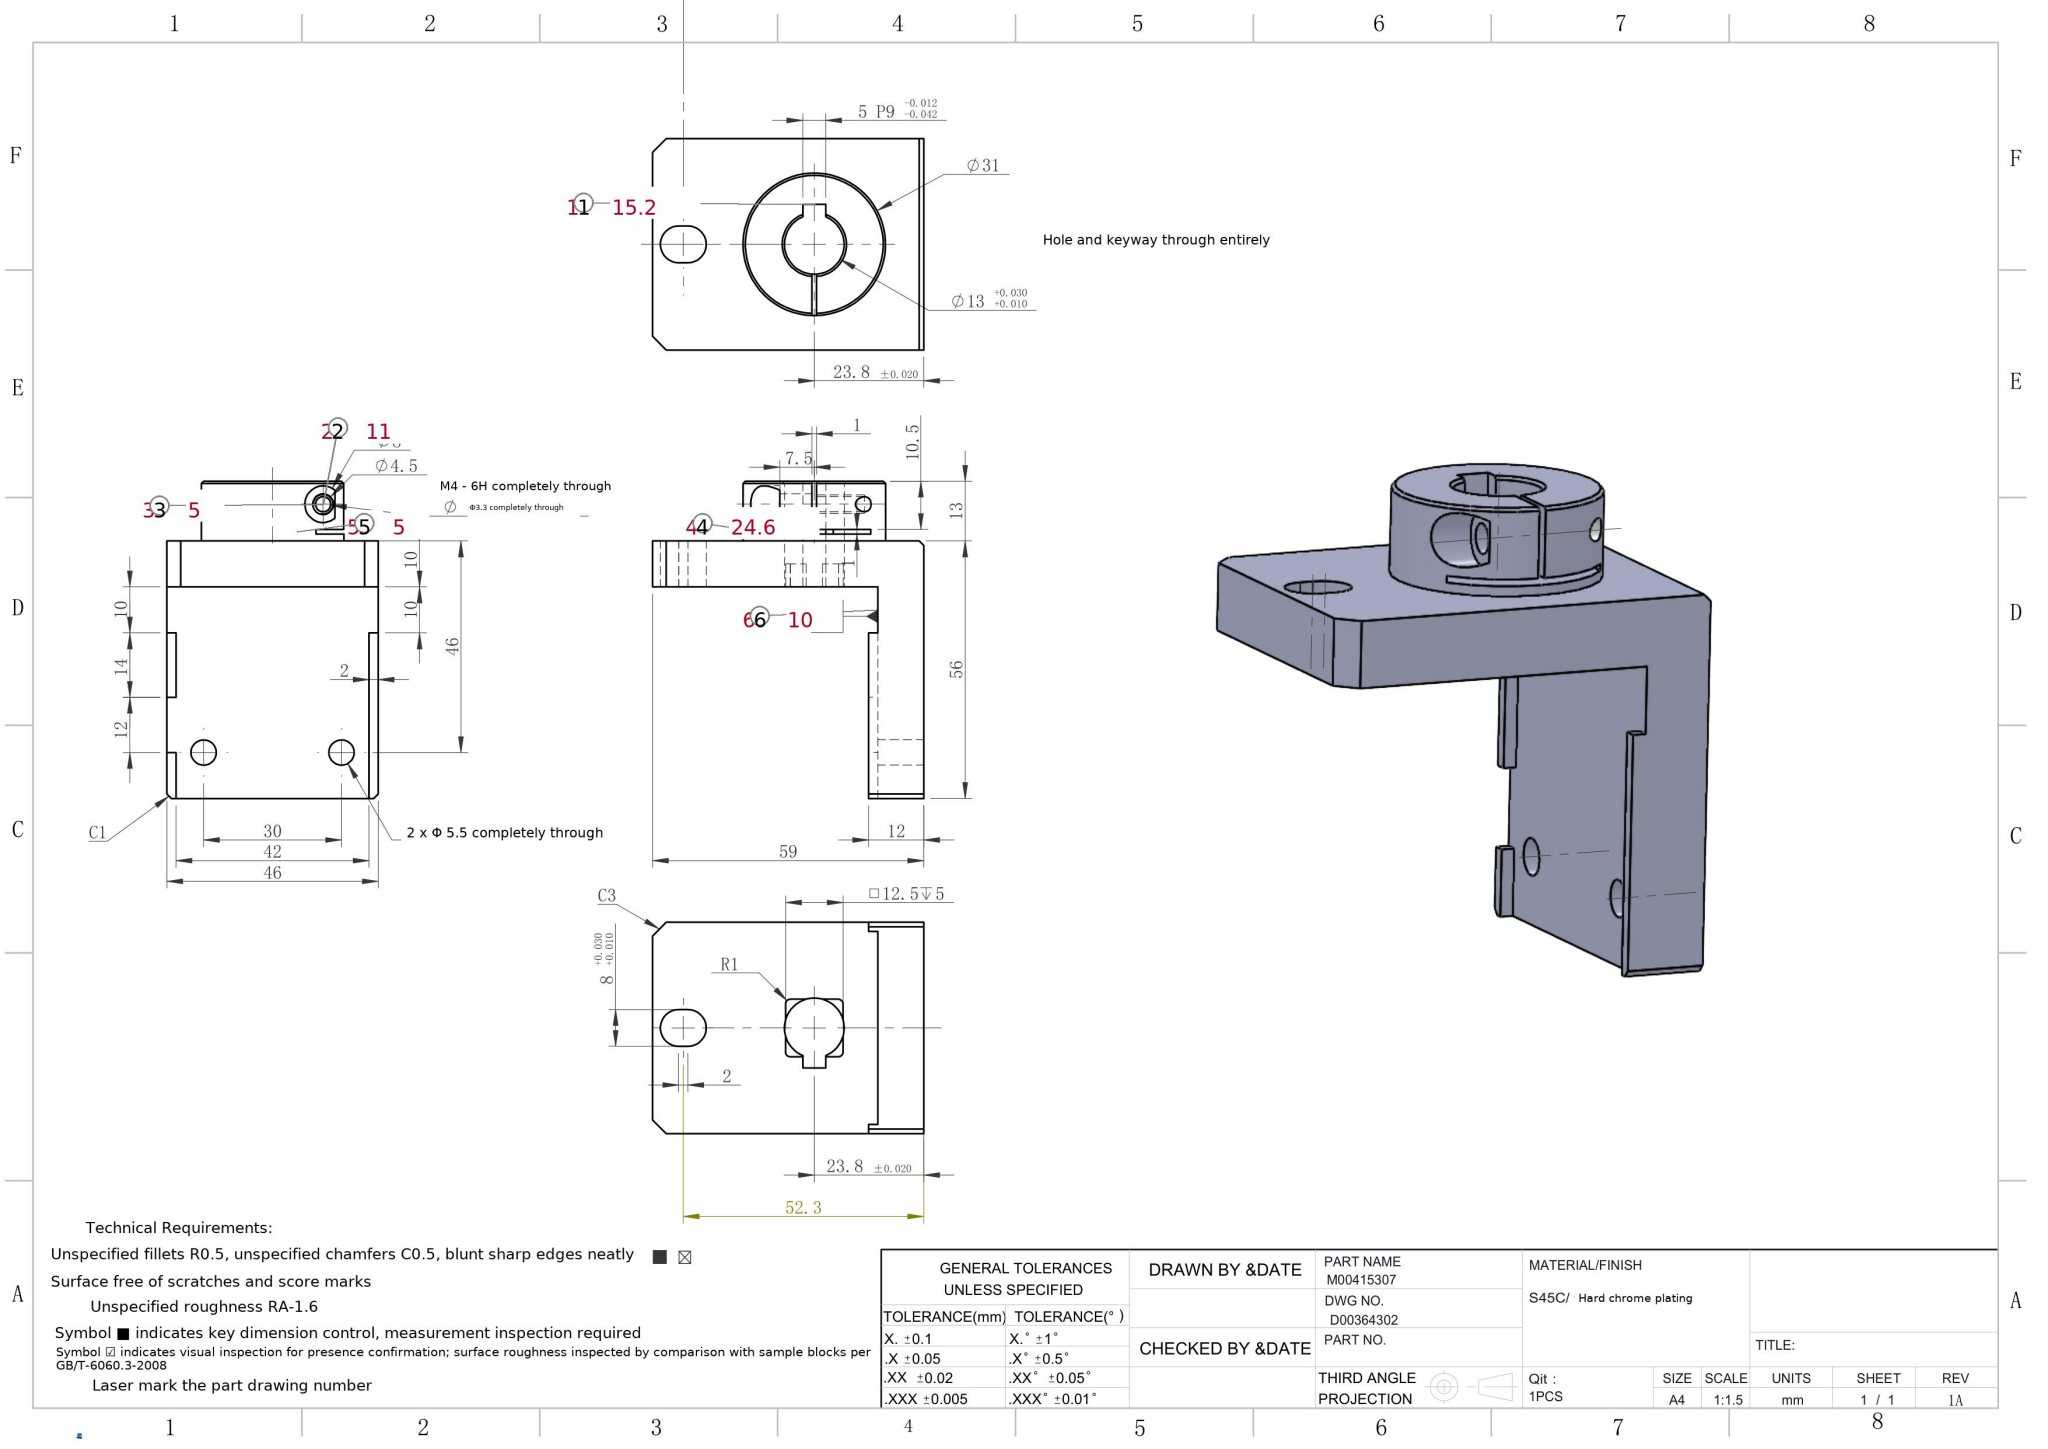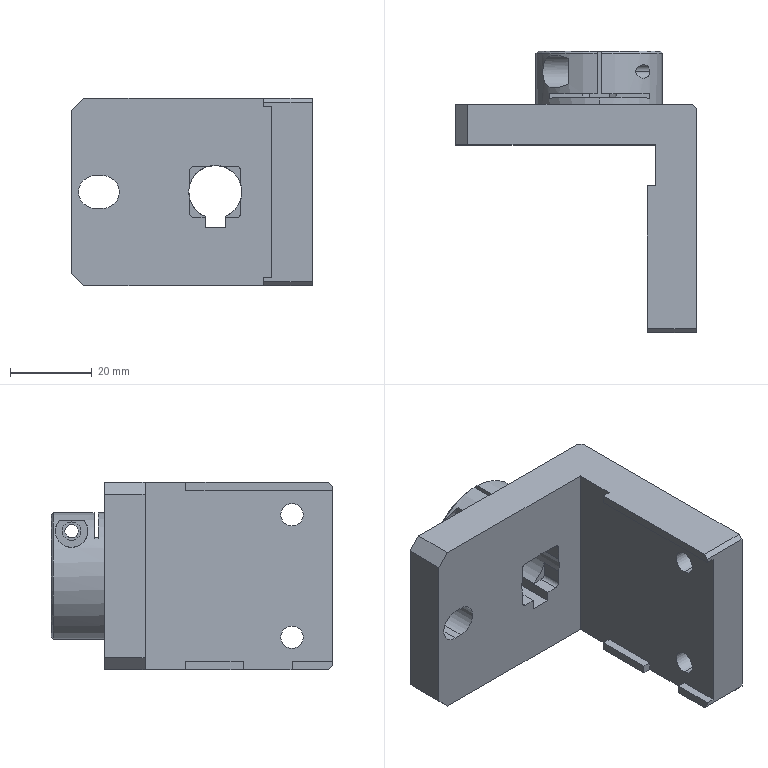Part | SolidWorks | mm | material S45C/ Hard chrome plating | 1 solid | 74 faces | box 59 x 69 x 46 mm | volume 52966 mm3 | plane 51 | cylinder 19 | cone 4 | commonest cylinder face diameters 5.5 x4 2 x4 8 x3 3.3 x2 4.5 x2 13 x2 31 x2